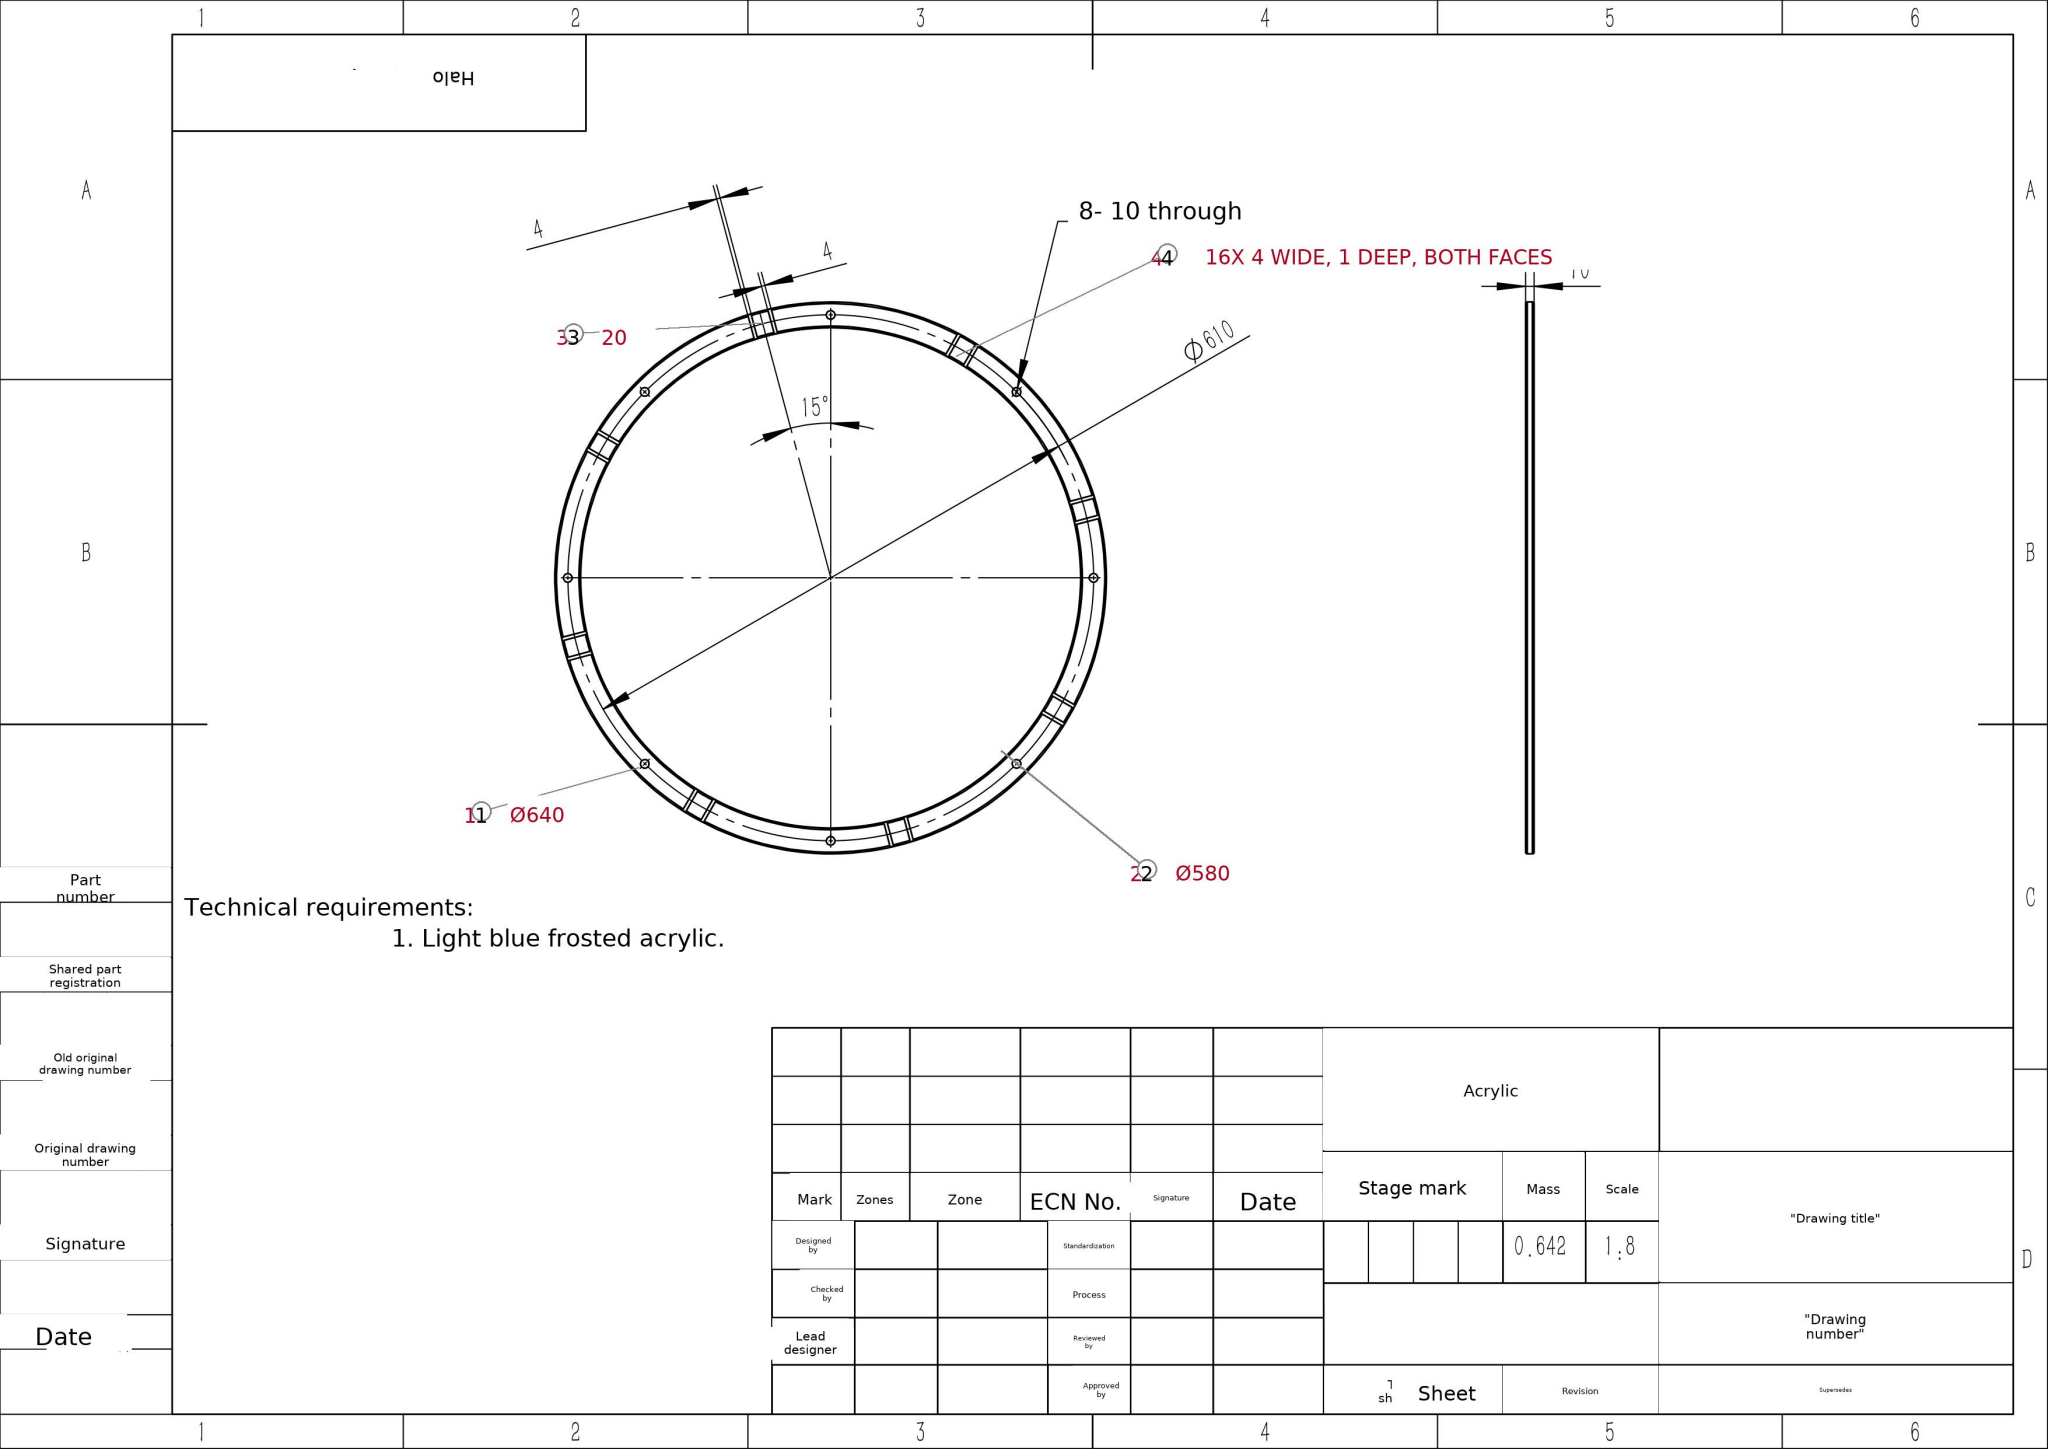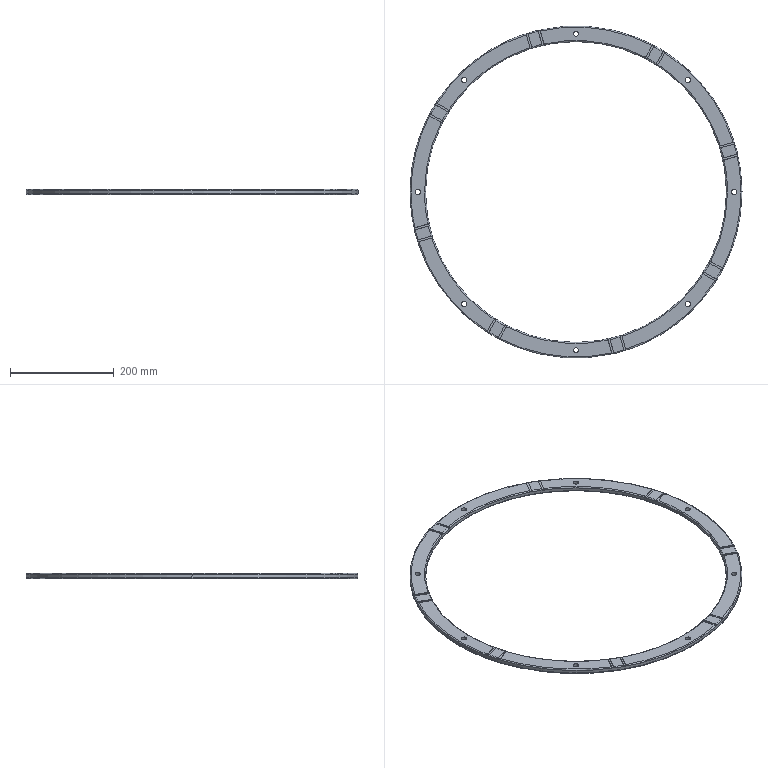Part | SolidWorks | mm | material Light blue frosted acrylic | 1 solid | 156 faces | box 640 x 640 x 10 mm | volume 558403 mm3 | plane 128 | cylinder 20 | torus 8 | commonest cylinder face diameters 10 x16 580 x2 640 x2
build123d program:
from build123d import *

# Parameters (mm, degrees)
SKETCH1_R                = 320
SKETCH1_R_2              = 290
BOSS_EXTRUDE1_DEPTH      = 5
FILLET1_R                = 2
SKETCH3_R                = 5
CUT_EXTRUDE2_DEPTH       = 39
CIRPATTERN2_COUNT        = 8
CUT_EXTRUDE3_DEPTH       = 1
CIRPATTERN3_COUNT        = 8
CIRPATTERN3_COPY_1_DEPTH = 1
CIRPATTERN3_COPY_2_DEPTH = 1
CIRPATTERN3_COPY_3_DEPTH = 1
CIRPATTERN3_COPY_4_DEPTH = 1
CIRPATTERN3_COPY_5_DEPTH = 1
CIRPATTERN3_COPY_6_DEPTH = 1
CIRPATTERN3_COPY_7_DEPTH = 1


with BuildPart() as part:
    # Sketch1 → Boss-Extrude1 (new, symmetric)
    with BuildSketch(Plane.XY):
        Circle(SKETCH1_R)
        Circle(SKETCH1_R_2, mode=Mode.SUBTRACT)
    extrude(amount=BOSS_EXTRUDE1_DEPTH, both=True)

    # Fillet1
    fillet1_edges = [part.edges().sort_by_distance(p)[0] for p in [
        (-320, 0, -5),
        (-320, 0, 5),
        (-290, 0, -5),
        (-290, 0, 5),
    ]]
    fillet(fillet1_edges, radius=FILLET1_R)

    # Sketch3 → Cut-Extrude2 (cut)
    with BuildSketch(Plane.XY.offset(5)):
        with Locations((0, 305)):
            Circle(SKETCH3_R)
    cut_extrude2 = extrude(amount=-CUT_EXTRUDE2_DEPTH, mode=Mode.SUBTRACT)

    # CirPattern2: Cut-Extrude2 ×8 about axis
    cirpattern2_axis = Axis((0, 0, 0), (0, 0, 1))
    for i in range(1, CIRPATTERN2_COUNT):
        add(cut_extrude2.rotate(cirpattern2_axis, i * 360 / CIRPATTERN2_COUNT), mode=Mode.SUBTRACT)

    # Sketch4 → Cut-Extrude3 (cut)
    with BuildSketch(Plane(origin=(0, 0, -5), x_dir=(-1, 0, 0), z_dir=(0, 0, -1))):
        with BuildLine():
            ThreePointArc((61.965, 285.349), (63.92, 284.918), (65.872, 284.473))
            Line((65.872, 284.473), (72.604, 309.601))
            ThreePointArc((72.604, 309.601), (70.654, 310.052), (68.702, 310.49))
            Line((68.702, 310.49), (61.965, 285.349))
        make_face()
        with BuildLine():
            ThreePointArc((68.702, 310.49), (70.654, 310.052), (72.604, 309.601))
            Line((72.604, 309.601), (73.122, 311.533))
            ThreePointArc((73.122, 311.533), (71.173, 311.985), (69.22, 312.424))
            Line((69.22, 312.424), (68.702, 310.49))
        make_face()
        with BuildLine():
            ThreePointArc((61.447, 283.415), (63.402, 282.984), (65.354, 282.54))
            Line((65.354, 282.54), (65.872, 284.473))
            ThreePointArc((65.872, 284.473), (63.92, 284.918), (61.965, 285.349))
            Line((61.965, 285.349), (61.447, 283.415))
        make_face()
        with BuildLine():
            Line((91.923, 304.424), (85.19, 279.297))
            ThreePointArc((85.19, 279.297), (87.103, 278.706), (89.011, 278.103))
            Line((89.011, 278.103), (95.748, 303.243))
            ThreePointArc((95.748, 303.243), (93.837, 303.84), (91.923, 304.424))
        make_face()
        with BuildLine():
            Line((92.441, 306.357), (91.923, 304.424))
            ThreePointArc((91.923, 304.424), (93.837, 303.84), (95.748, 303.243))
            Line((95.748, 303.243), (96.266, 305.177))
            ThreePointArc((96.266, 305.177), (94.355, 305.773), (92.441, 306.357))
        make_face()
        with BuildLine():
            Line((85.19, 279.297), (84.672, 277.364))
            ThreePointArc((84.672, 277.364), (86.585, 276.773), (88.493, 276.168))
            Line((88.493, 276.168), (89.011, 278.103))
            ThreePointArc((89.011, 278.103), (87.103, 278.706), (85.19, 279.297))
        make_face()
    cut_extrude3 = extrude(amount=-CUT_EXTRUDE3_DEPTH, mode=Mode.SUBTRACT)

    # Mirror1: Cut-Extrude3 across plane
    add(cut_extrude3.mirror(Plane.XY), mode=Mode.SUBTRACT)

    # CirPattern3: Cut-Extrude3 ×8 about axis
    cirpattern3_axis = Axis((0, 0, 0), (0, 0, 1))
    for i in range(1, CIRPATTERN3_COUNT):
        add(cut_extrude3.rotate(cirpattern3_axis, i * 360 / CIRPATTERN3_COUNT), mode=Mode.SUBTRACT)

    # CirPattern3 copy 1 sketch → CirPattern3 copy 1 (cut)
    with BuildSketch(Plane(origin=(0, 0, 5), x_dir=(-0.7071, -0.7071, 0), z_dir=(0, 0, 1))):
        with BuildLine():
            ThreePointArc((61.965, -285.349), (63.92, -284.918), (65.872, -284.473))
            Line((65.872, -284.473), (72.604, -309.601))
            ThreePointArc((72.604, -309.601), (70.654, -310.052), (68.702, -310.49))
            Line((68.702, -310.49), (61.965, -285.349))
        make_face()
        with BuildLine():
            ThreePointArc((68.702, -310.49), (70.654, -310.052), (72.604, -309.601))
            Line((72.604, -309.601), (73.122, -311.533))
            ThreePointArc((73.122, -311.533), (71.173, -311.985), (69.22, -312.424))
            Line((69.22, -312.424), (68.702, -310.49))
        make_face()
        with BuildLine():
            ThreePointArc((61.447, -283.415), (63.402, -282.984), (65.354, -282.54))
            Line((65.354, -282.54), (65.872, -284.473))
            ThreePointArc((65.872, -284.473), (63.92, -284.918), (61.965, -285.349))
            Line((61.965, -285.349), (61.447, -283.415))
        make_face()
        with BuildLine():
            Line((91.923, -304.424), (85.19, -279.297))
            ThreePointArc((85.19, -279.297), (87.103, -278.706), (89.011, -278.103))
            Line((89.011, -278.103), (95.748, -303.243))
            ThreePointArc((95.748, -303.243), (93.837, -303.84), (91.923, -304.424))
        make_face()
        with BuildLine():
            Line((92.441, -306.357), (91.923, -304.424))
            ThreePointArc((91.923, -304.424), (93.837, -303.84), (95.748, -303.243))
            Line((95.748, -303.243), (96.266, -305.177))
            ThreePointArc((96.266, -305.177), (94.355, -305.773), (92.441, -306.357))
        make_face()
        with BuildLine():
            Line((85.19, -279.297), (84.672, -277.364))
            ThreePointArc((84.672, -277.364), (86.585, -276.773), (88.493, -276.168))
            Line((88.493, -276.168), (89.011, -278.103))
            ThreePointArc((89.011, -278.103), (87.103, -278.706), (85.19, -279.297))
        make_face()
    extrude(amount=-CIRPATTERN3_COPY_1_DEPTH, mode=Mode.SUBTRACT)

    # CirPattern3 copy 2 sketch → CirPattern3 copy 2 (cut)
    with BuildSketch(Plane(origin=(0, 0, 5), x_dir=(0, -1, 0), z_dir=(0, 0, 1))):
        with BuildLine():
            ThreePointArc((61.965, -285.349), (63.92, -284.918), (65.872, -284.473))
            Line((65.872, -284.473), (72.604, -309.601))
            ThreePointArc((72.604, -309.601), (70.654, -310.052), (68.702, -310.49))
            Line((68.702, -310.49), (61.965, -285.349))
        make_face()
        with BuildLine():
            ThreePointArc((68.702, -310.49), (70.654, -310.052), (72.604, -309.601))
            Line((72.604, -309.601), (73.122, -311.533))
            ThreePointArc((73.122, -311.533), (71.173, -311.985), (69.22, -312.424))
            Line((69.22, -312.424), (68.702, -310.49))
        make_face()
        with BuildLine():
            ThreePointArc((61.447, -283.415), (63.402, -282.984), (65.354, -282.54))
            Line((65.354, -282.54), (65.872, -284.473))
            ThreePointArc((65.872, -284.473), (63.92, -284.918), (61.965, -285.349))
            Line((61.965, -285.349), (61.447, -283.415))
        make_face()
        with BuildLine():
            Line((91.923, -304.424), (85.19, -279.297))
            ThreePointArc((85.19, -279.297), (87.103, -278.706), (89.011, -278.103))
            Line((89.011, -278.103), (95.748, -303.243))
            ThreePointArc((95.748, -303.243), (93.837, -303.84), (91.923, -304.424))
        make_face()
        with BuildLine():
            Line((92.441, -306.357), (91.923, -304.424))
            ThreePointArc((91.923, -304.424), (93.837, -303.84), (95.748, -303.243))
            Line((95.748, -303.243), (96.266, -305.177))
            ThreePointArc((96.266, -305.177), (94.355, -305.773), (92.441, -306.357))
        make_face()
        with BuildLine():
            Line((85.19, -279.297), (84.672, -277.364))
            ThreePointArc((84.672, -277.364), (86.585, -276.773), (88.493, -276.168))
            Line((88.493, -276.168), (89.011, -278.103))
            ThreePointArc((89.011, -278.103), (87.103, -278.706), (85.19, -279.297))
        make_face()
    extrude(amount=-CIRPATTERN3_COPY_2_DEPTH, mode=Mode.SUBTRACT)

    # CirPattern3 copy 3 sketch → CirPattern3 copy 3 (cut)
    with BuildSketch(Plane(origin=(0, 0, 5), x_dir=(0.7071, -0.7071, 0), z_dir=(0, 0, 1))):
        with BuildLine():
            ThreePointArc((61.965, -285.349), (63.92, -284.918), (65.872, -284.473))
            Line((65.872, -284.473), (72.604, -309.601))
            ThreePointArc((72.604, -309.601), (70.654, -310.052), (68.702, -310.49))
            Line((68.702, -310.49), (61.965, -285.349))
        make_face()
        with BuildLine():
            ThreePointArc((68.702, -310.49), (70.654, -310.052), (72.604, -309.601))
            Line((72.604, -309.601), (73.122, -311.533))
            ThreePointArc((73.122, -311.533), (71.173, -311.985), (69.22, -312.424))
            Line((69.22, -312.424), (68.702, -310.49))
        make_face()
        with BuildLine():
            ThreePointArc((61.447, -283.415), (63.402, -282.984), (65.354, -282.54))
            Line((65.354, -282.54), (65.872, -284.473))
            ThreePointArc((65.872, -284.473), (63.92, -284.918), (61.965, -285.349))
            Line((61.965, -285.349), (61.447, -283.415))
        make_face()
        with BuildLine():
            Line((91.923, -304.424), (85.19, -279.297))
            ThreePointArc((85.19, -279.297), (87.103, -278.706), (89.011, -278.103))
            Line((89.011, -278.103), (95.748, -303.243))
            ThreePointArc((95.748, -303.243), (93.837, -303.84), (91.923, -304.424))
        make_face()
        with BuildLine():
            Line((92.441, -306.357), (91.923, -304.424))
            ThreePointArc((91.923, -304.424), (93.837, -303.84), (95.748, -303.243))
            Line((95.748, -303.243), (96.266, -305.177))
            ThreePointArc((96.266, -305.177), (94.355, -305.773), (92.441, -306.357))
        make_face()
        with BuildLine():
            Line((85.19, -279.297), (84.672, -277.364))
            ThreePointArc((84.672, -277.364), (86.585, -276.773), (88.493, -276.168))
            Line((88.493, -276.168), (89.011, -278.103))
            ThreePointArc((89.011, -278.103), (87.103, -278.706), (85.19, -279.297))
        make_face()
    extrude(amount=-CIRPATTERN3_COPY_3_DEPTH, mode=Mode.SUBTRACT)

    # CirPattern3 copy 4 sketch → CirPattern3 copy 4 (cut)
    with BuildSketch(Plane.XY.offset(5)):
        with BuildLine():
            ThreePointArc((61.965, -285.349), (63.92, -284.918), (65.872, -284.473))
            Line((65.872, -284.473), (72.604, -309.601))
            ThreePointArc((72.604, -309.601), (70.654, -310.052), (68.702, -310.49))
            Line((68.702, -310.49), (61.965, -285.349))
        make_face()
        with BuildLine():
            ThreePointArc((68.702, -310.49), (70.654, -310.052), (72.604, -309.601))
            Line((72.604, -309.601), (73.122, -311.533))
            ThreePointArc((73.122, -311.533), (71.173, -311.985), (69.22, -312.424))
            Line((69.22, -312.424), (68.702, -310.49))
        make_face()
        with BuildLine():
            ThreePointArc((61.447, -283.415), (63.402, -282.984), (65.354, -282.54))
            Line((65.354, -282.54), (65.872, -284.473))
            ThreePointArc((65.872, -284.473), (63.92, -284.918), (61.965, -285.349))
            Line((61.965, -285.349), (61.447, -283.415))
        make_face()
        with BuildLine():
            Line((91.923, -304.424), (85.19, -279.297))
            ThreePointArc((85.19, -279.297), (87.103, -278.706), (89.011, -278.103))
            Line((89.011, -278.103), (95.748, -303.243))
            ThreePointArc((95.748, -303.243), (93.837, -303.84), (91.923, -304.424))
        make_face()
        with BuildLine():
            Line((92.441, -306.357), (91.923, -304.424))
            ThreePointArc((91.923, -304.424), (93.837, -303.84), (95.748, -303.243))
            Line((95.748, -303.243), (96.266, -305.177))
            ThreePointArc((96.266, -305.177), (94.355, -305.773), (92.441, -306.357))
        make_face()
        with BuildLine():
            Line((85.19, -279.297), (84.672, -277.364))
            ThreePointArc((84.672, -277.364), (86.585, -276.773), (88.493, -276.168))
            Line((88.493, -276.168), (89.011, -278.103))
            ThreePointArc((89.011, -278.103), (87.103, -278.706), (85.19, -279.297))
        make_face()
    extrude(amount=-CIRPATTERN3_COPY_4_DEPTH, mode=Mode.SUBTRACT)

    # CirPattern3 copy 5 sketch → CirPattern3 copy 5 (cut)
    with BuildSketch(Plane(origin=(0, 0, 5), x_dir=(0.7071, 0.7071, 0), z_dir=(0, 0, 1))):
        with BuildLine():
            ThreePointArc((61.965, -285.349), (63.92, -284.918), (65.872, -284.473))
            Line((65.872, -284.473), (72.604, -309.601))
            ThreePointArc((72.604, -309.601), (70.654, -310.052), (68.702, -310.49))
            Line((68.702, -310.49), (61.965, -285.349))
        make_face()
        with BuildLine():
            ThreePointArc((68.702, -310.49), (70.654, -310.052), (72.604, -309.601))
            Line((72.604, -309.601), (73.122, -311.533))
            ThreePointArc((73.122, -311.533), (71.173, -311.985), (69.22, -312.424))
            Line((69.22, -312.424), (68.702, -310.49))
        make_face()
        with BuildLine():
            ThreePointArc((61.447, -283.415), (63.402, -282.984), (65.354, -282.54))
            Line((65.354, -282.54), (65.872, -284.473))
            ThreePointArc((65.872, -284.473), (63.92, -284.918), (61.965, -285.349))
            Line((61.965, -285.349), (61.447, -283.415))
        make_face()
        with BuildLine():
            Line((91.923, -304.424), (85.19, -279.297))
            ThreePointArc((85.19, -279.297), (87.103, -278.706), (89.011, -278.103))
            Line((89.011, -278.103), (95.748, -303.243))
            ThreePointArc((95.748, -303.243), (93.837, -303.84), (91.923, -304.424))
        make_face()
        with BuildLine():
            Line((92.441, -306.357), (91.923, -304.424))
            ThreePointArc((91.923, -304.424), (93.837, -303.84), (95.748, -303.243))
            Line((95.748, -303.243), (96.266, -305.177))
            ThreePointArc((96.266, -305.177), (94.355, -305.773), (92.441, -306.357))
        make_face()
        with BuildLine():
            Line((85.19, -279.297), (84.672, -277.364))
            ThreePointArc((84.672, -277.364), (86.585, -276.773), (88.493, -276.168))
            Line((88.493, -276.168), (89.011, -278.103))
            ThreePointArc((89.011, -278.103), (87.103, -278.706), (85.19, -279.297))
        make_face()
    extrude(amount=-CIRPATTERN3_COPY_5_DEPTH, mode=Mode.SUBTRACT)

    # CirPattern3 copy 6 sketch → CirPattern3 copy 6 (cut)
    with BuildSketch(Plane(origin=(0, 0, 5), x_dir=(0, 1, 0), z_dir=(0, 0, 1))):
        with BuildLine():
            ThreePointArc((61.965, -285.349), (63.92, -284.918), (65.872, -284.473))
            Line((65.872, -284.473), (72.604, -309.601))
            ThreePointArc((72.604, -309.601), (70.654, -310.052), (68.702, -310.49))
            Line((68.702, -310.49), (61.965, -285.349))
        make_face()
        with BuildLine():
            ThreePointArc((68.702, -310.49), (70.654, -310.052), (72.604, -309.601))
            Line((72.604, -309.601), (73.122, -311.533))
            ThreePointArc((73.122, -311.533), (71.173, -311.985), (69.22, -312.424))
            Line((69.22, -312.424), (68.702, -310.49))
        make_face()
        with BuildLine():
            ThreePointArc((61.447, -283.415), (63.402, -282.984), (65.354, -282.54))
            Line((65.354, -282.54), (65.872, -284.473))
            ThreePointArc((65.872, -284.473), (63.92, -284.918), (61.965, -285.349))
            Line((61.965, -285.349), (61.447, -283.415))
        make_face()
        with BuildLine():
            Line((91.923, -304.424), (85.19, -279.297))
            ThreePointArc((85.19, -279.297), (87.103, -278.706), (89.011, -278.103))
            Line((89.011, -278.103), (95.748, -303.243))
            ThreePointArc((95.748, -303.243), (93.837, -303.84), (91.923, -304.424))
        make_face()
        with BuildLine():
            Line((92.441, -306.357), (91.923, -304.424))
            ThreePointArc((91.923, -304.424), (93.837, -303.84), (95.748, -303.243))
            Line((95.748, -303.243), (96.266, -305.177))
            ThreePointArc((96.266, -305.177), (94.355, -305.773), (92.441, -306.357))
        make_face()
        with BuildLine():
            Line((85.19, -279.297), (84.672, -277.364))
            ThreePointArc((84.672, -277.364), (86.585, -276.773), (88.493, -276.168))
            Line((88.493, -276.168), (89.011, -278.103))
            ThreePointArc((89.011, -278.103), (87.103, -278.706), (85.19, -279.297))
        make_face()
    extrude(amount=-CIRPATTERN3_COPY_6_DEPTH, mode=Mode.SUBTRACT)

    # CirPattern3 copy 7 sketch → CirPattern3 copy 7 (cut)
    with BuildSketch(Plane(origin=(0, 0, 5), x_dir=(-0.7071, 0.7071, 0), z_dir=(0, 0, 1))):
        with BuildLine():
            ThreePointArc((61.965, -285.349), (63.92, -284.918), (65.872, -284.473))
            Line((65.872, -284.473), (72.604, -309.601))
            ThreePointArc((72.604, -309.601), (70.654, -310.052), (68.702, -310.49))
            Line((68.702, -310.49), (61.965, -285.349))
        make_face()
        with BuildLine():
            ThreePointArc((68.702, -310.49), (70.654, -310.052), (72.604, -309.601))
            Line((72.604, -309.601), (73.122, -311.533))
            ThreePointArc((73.122, -311.533), (71.173, -311.985), (69.22, -312.424))
            Line((69.22, -312.424), (68.702, -310.49))
        make_face()
        with BuildLine():
            ThreePointArc((61.447, -283.415), (63.402, -282.984), (65.354, -282.54))
            Line((65.354, -282.54), (65.872, -284.473))
            ThreePointArc((65.872, -284.473), (63.92, -284.918), (61.965, -285.349))
            Line((61.965, -285.349), (61.447, -283.415))
        make_face()
        with BuildLine():
            Line((91.923, -304.424), (85.19, -279.297))
            ThreePointArc((85.19, -279.297), (87.103, -278.706), (89.011, -278.103))
            Line((89.011, -278.103), (95.748, -303.243))
            ThreePointArc((95.748, -303.243), (93.837, -303.84), (91.923, -304.424))
        make_face()
        with BuildLine():
            Line((92.441, -306.357), (91.923, -304.424))
            ThreePointArc((91.923, -304.424), (93.837, -303.84), (95.748, -303.243))
            Line((95.748, -303.243), (96.266, -305.177))
            ThreePointArc((96.266, -305.177), (94.355, -305.773), (92.441, -306.357))
        make_face()
        with BuildLine():
            Line((85.19, -279.297), (84.672, -277.364))
            ThreePointArc((84.672, -277.364), (86.585, -276.773), (88.493, -276.168))
            Line((88.493, -276.168), (89.011, -278.103))
            ThreePointArc((89.011, -278.103), (87.103, -278.706), (85.19, -279.297))
        make_face()
    extrude(amount=-CIRPATTERN3_COPY_7_DEPTH, mode=Mode.SUBTRACT)


solid = part.part